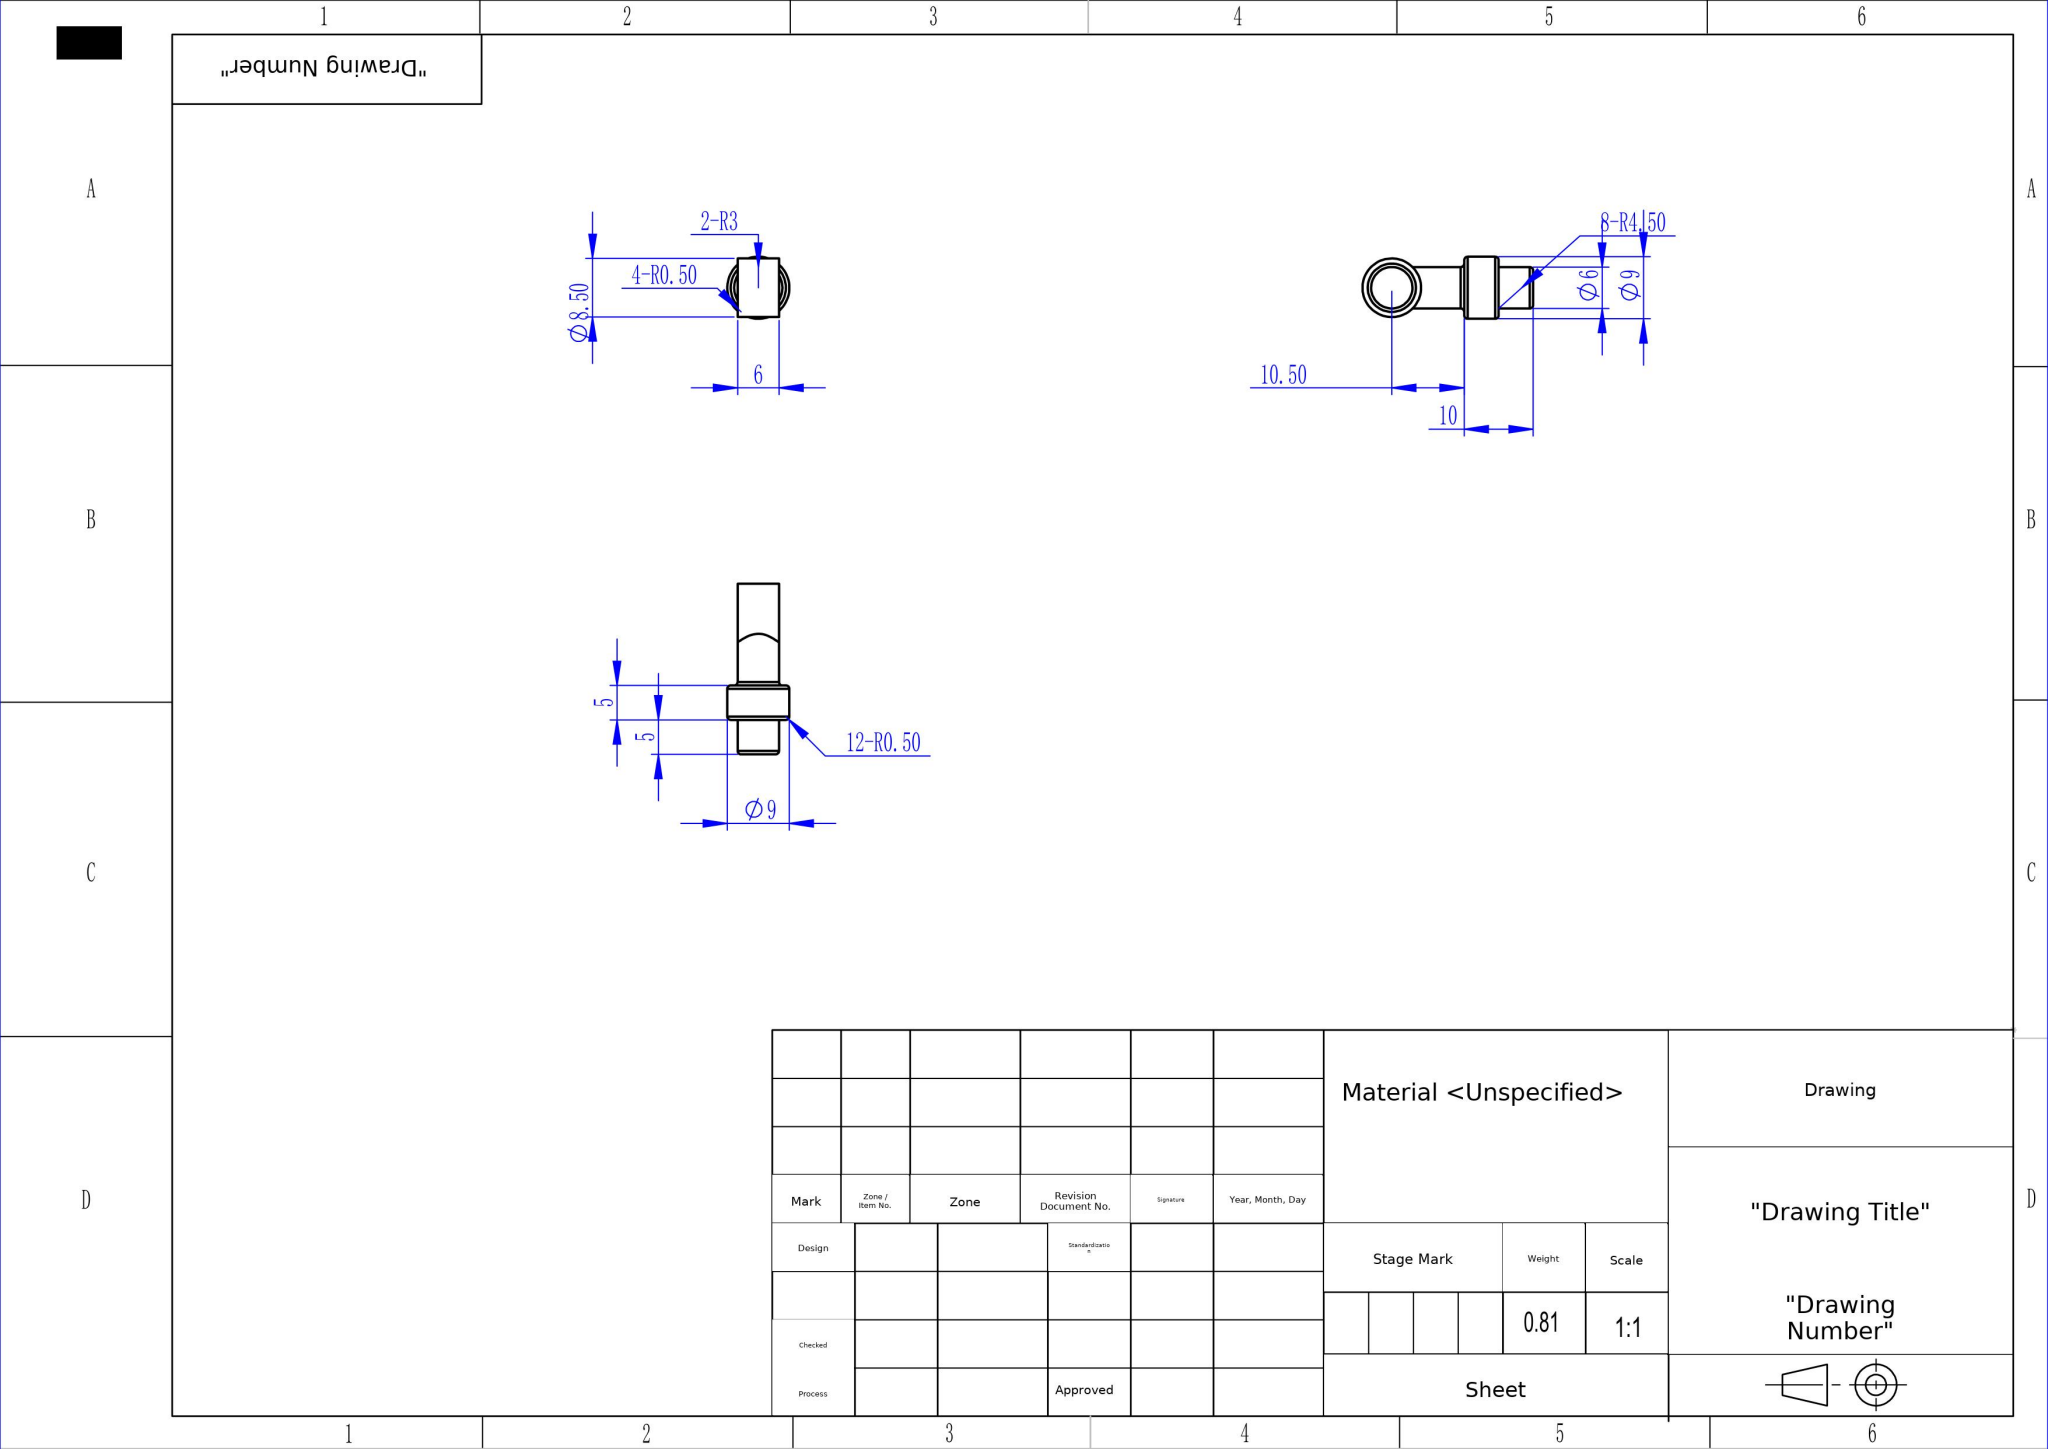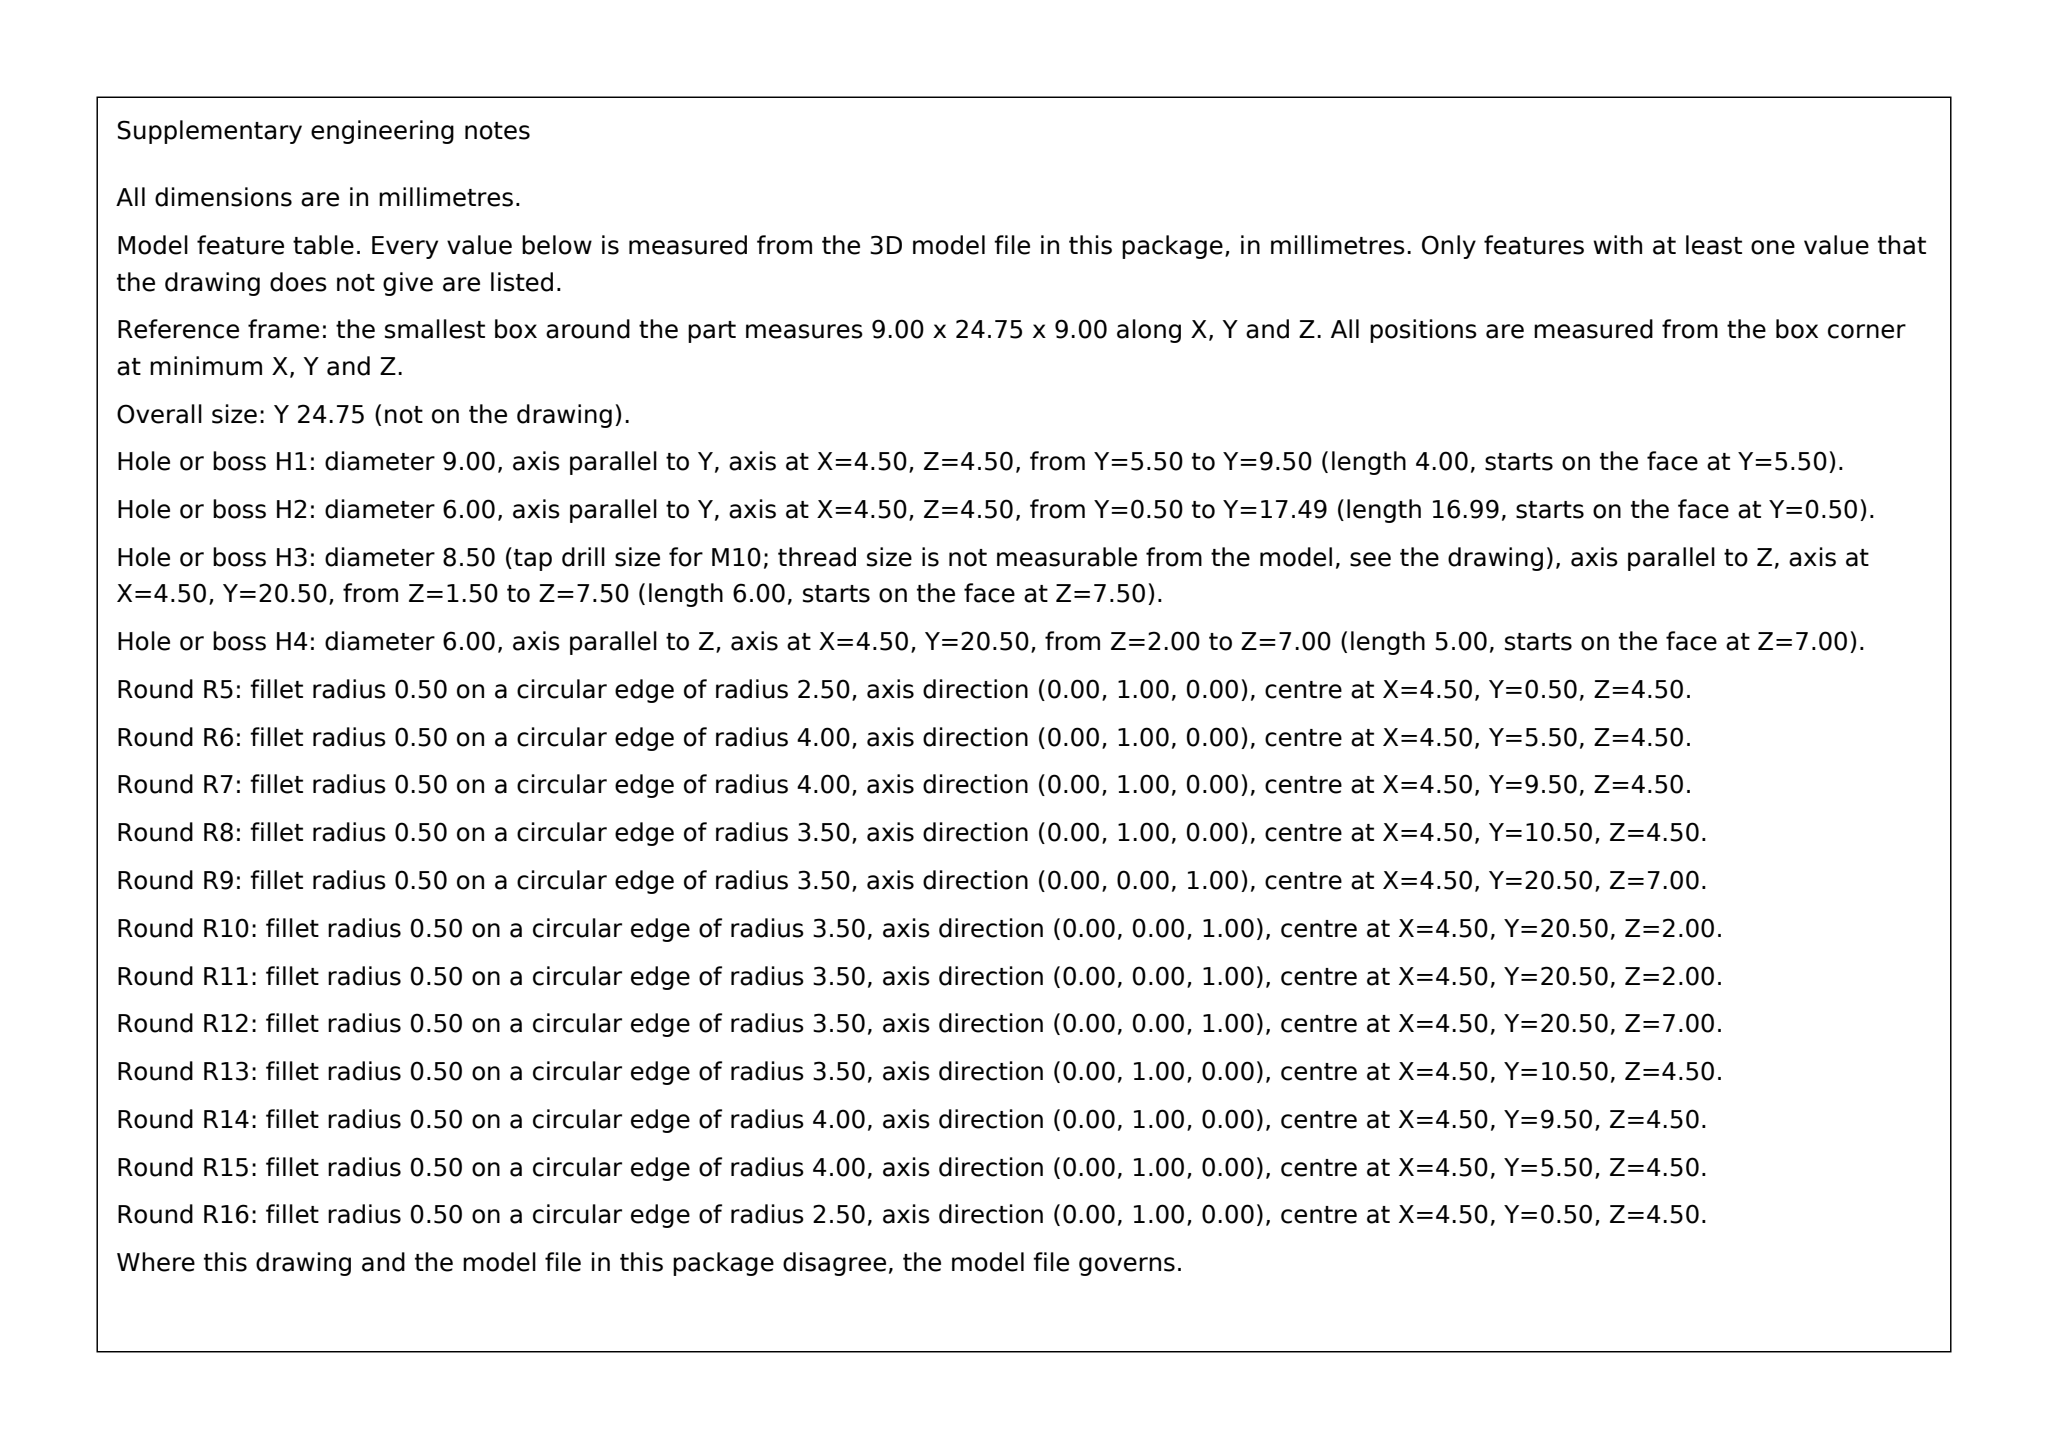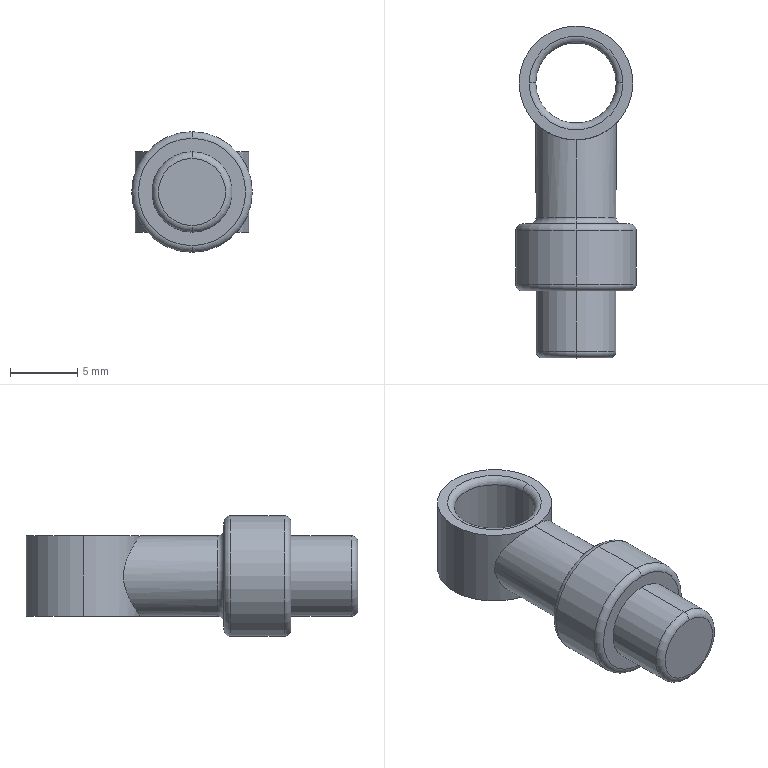Part | SolidWorks | mm | 1 solid | 28 faces | box 9 x 24.75 x 9 mm | volume 810 mm3 | torus 12 | cylinder 11 | plane 5 | commonest cylinder face diameters 6 x6 8.5 x3 9 x2
STEP:
#1=CARTESIAN_POINT('',(0.,0.,-2.5));
#2=VERTEX_POINT('',#1);
#3=CARTESIAN_POINT('',(0.,0.,2.5));
#4=VERTEX_POINT('',#3);
#5=CARTESIAN_POINT('',(0.,0.,0.));
#6=DIRECTION('',(0.,-1.,0.));
#7=DIRECTION('',(0.,0.,1.));
#8=AXIS2_PLACEMENT_3D('',#5,#6,#7);
#9=CIRCLE('',#8,2.5);
#10=EDGE_CURVE('',#2,#4,#9,.T.);
#11=ORIENTED_EDGE('',*,*,#10,.F.);
#12=CARTESIAN_POINT('',(0.,0.5,-3.));
#13=VERTEX_POINT('',#12);
#14=CARTESIAN_POINT('',(0.,0.5,-2.5));
#15=DIRECTION('',(1.,0.,0.));
#16=DIRECTION('',(0.,0.,-1.));
#17=AXIS2_PLACEMENT_3D('',#14,#15,#16);
#18=CIRCLE('',#17,0.5);
#19=EDGE_CURVE('',#2,#13,#18,.T.);
#20=ORIENTED_EDGE('',*,*,#19,.T.);
#21=CARTESIAN_POINT('',(0.,0.5,3.));
#22=VERTEX_POINT('',#21);
#23=CARTESIAN_POINT('',(0.,0.5,0.));
#24=DIRECTION('',(0.,1.,0.));
#25=DIRECTION('',(0.,0.,1.));
#26=AXIS2_PLACEMENT_3D('',#23,#24,#25);
#27=CIRCLE('',#26,3.);
#28=EDGE_CURVE('',#22,#13,#27,.T.);
#29=ORIENTED_EDGE('',*,*,#28,.F.);
#30=CARTESIAN_POINT('',(0.,0.5,2.5));
#31=DIRECTION('',(-1.,0.,0.));
#32=DIRECTION('',(0.,0.,1.));
#33=AXIS2_PLACEMENT_3D('',#30,#31,#32);
#34=CIRCLE('',#33,0.5);
#35=EDGE_CURVE('',#4,#22,#34,.T.);
#36=ORIENTED_EDGE('',*,*,#35,.F.);
#37=EDGE_LOOP('',(#11,#20,#29,#36));
#38=FACE_OUTER_BOUND('',#37,.T.);
#39=CARTESIAN_POINT('',(0.,0.5,0.));
#40=DIRECTION('',(0.,1.,0.));
#41=DIRECTION('',(0.,0.,1.));
#42=AXIS2_PLACEMENT_3D('',#39,#40,#41);
#43=TOROIDAL_SURFACE('',#42,2.5,0.5);
#44=ADVANCED_FACE('',(#38),#43,.T.);
#45=CARTESIAN_POINT('',(0.,5.,-4.));
#46=VERTEX_POINT('',#45);
#47=CARTESIAN_POINT('',(0.,5.,4.));
#48=VERTEX_POINT('',#47);
#49=CARTESIAN_POINT('',(0.,5.,0.));
#50=DIRECTION('',(0.,-1.,0.));
#51=DIRECTION('',(0.,0.,1.));
#52=AXIS2_PLACEMENT_3D('',#49,#50,#51);
#53=CIRCLE('',#52,4.);
#54=EDGE_CURVE('',#46,#48,#53,.T.);
#55=ORIENTED_EDGE('',*,*,#54,.F.);
#56=CARTESIAN_POINT('',(0.,5.5,-4.5));
#57=VERTEX_POINT('',#56);
#58=CARTESIAN_POINT('',(0.,5.5,-4.));
#59=DIRECTION('',(1.,0.,0.));
#60=DIRECTION('',(0.,0.,-1.));
#61=AXIS2_PLACEMENT_3D('',#58,#59,#60);
#62=CIRCLE('',#61,0.5);
#63=EDGE_CURVE('',#46,#57,#62,.T.);
#64=ORIENTED_EDGE('',*,*,#63,.T.);
#65=CARTESIAN_POINT('',(0.,5.5,4.5));
#66=VERTEX_POINT('',#65);
#67=CARTESIAN_POINT('',(0.,5.5,0.));
#68=DIRECTION('',(0.,1.,0.));
#69=DIRECTION('',(0.,0.,1.));
#70=AXIS2_PLACEMENT_3D('',#67,#68,#69);
#71=CIRCLE('',#70,4.5);
#72=EDGE_CURVE('',#66,#57,#71,.T.);
#73=ORIENTED_EDGE('',*,*,#72,.F.);
#74=CARTESIAN_POINT('',(0.,5.5,4.));
#75=DIRECTION('',(-1.,0.,0.));
#76=DIRECTION('',(0.,0.,1.));
#77=AXIS2_PLACEMENT_3D('',#74,#75,#76);
#78=CIRCLE('',#77,0.5);
#79=EDGE_CURVE('',#48,#66,#78,.T.);
#80=ORIENTED_EDGE('',*,*,#79,.F.);
#81=EDGE_LOOP('',(#55,#64,#73,#80));
#82=FACE_OUTER_BOUND('',#81,.T.);
#83=CARTESIAN_POINT('',(0.,5.5,0.));
#84=DIRECTION('',(0.,1.,0.));
#85=DIRECTION('',(0.,0.,1.));
#86=AXIS2_PLACEMENT_3D('',#83,#84,#85);
#87=TOROIDAL_SURFACE('',#86,4.,0.5);
#88=ADVANCED_FACE('',(#82),#87,.T.);
#89=CARTESIAN_POINT('',(0.,9.5,-4.5));
#90=VERTEX_POINT('',#89);
#91=CARTESIAN_POINT('',(0.,9.5,4.5));
#92=VERTEX_POINT('',#91);
#93=CARTESIAN_POINT('',(0.,9.5,0.));
#94=DIRECTION('',(0.,-1.,0.));
#95=DIRECTION('',(0.,0.,1.));
#96=AXIS2_PLACEMENT_3D('',#93,#94,#95);
#97=CIRCLE('',#96,4.5);
#98=EDGE_CURVE('',#90,#92,#97,.T.);
#99=ORIENTED_EDGE('',*,*,#98,.F.);
#100=CARTESIAN_POINT('',(0.,10.,-4.));
#101=VERTEX_POINT('',#100);
#102=CARTESIAN_POINT('',(0.,9.5,-4.));
#103=DIRECTION('',(1.,0.,0.));
#104=DIRECTION('',(0.,0.,-1.));
#105=AXIS2_PLACEMENT_3D('',#102,#103,#104);
#106=CIRCLE('',#105,0.5);
#107=EDGE_CURVE('',#90,#101,#106,.T.);
#108=ORIENTED_EDGE('',*,*,#107,.T.);
#109=CARTESIAN_POINT('',(0.,10.,4.));
#110=VERTEX_POINT('',#109);
#111=CARTESIAN_POINT('',(0.,10.,0.));
#112=DIRECTION('',(0.,1.,0.));
#113=DIRECTION('',(0.,0.,1.));
#114=AXIS2_PLACEMENT_3D('',#111,#112,#113);
#115=CIRCLE('',#114,4.);
#116=EDGE_CURVE('',#110,#101,#115,.T.);
#117=ORIENTED_EDGE('',*,*,#116,.F.);
#118=CARTESIAN_POINT('',(0.,9.5,4.));
#119=DIRECTION('',(-1.,0.,0.));
#120=DIRECTION('',(0.,0.,1.));
#121=AXIS2_PLACEMENT_3D('',#118,#119,#120);
#122=CIRCLE('',#121,0.5);
#123=EDGE_CURVE('',#92,#110,#122,.T.);
#124=ORIENTED_EDGE('',*,*,#123,.F.);
#125=EDGE_LOOP('',(#99,#108,#117,#124));
#126=FACE_OUTER_BOUND('',#125,.T.);
#127=CARTESIAN_POINT('',(0.,9.5,0.));
#128=DIRECTION('',(0.,1.,0.));
#129=DIRECTION('',(0.,0.,1.));
#130=AXIS2_PLACEMENT_3D('',#127,#128,#129);
#131=TOROIDAL_SURFACE('',#130,4.,0.5);
#132=ADVANCED_FACE('',(#126),#131,.T.);
#133=CARTESIAN_POINT('',(0.,10.5,-3.));
#134=VERTEX_POINT('',#133);
#135=CARTESIAN_POINT('',(0.,10.5,3.));
#136=VERTEX_POINT('',#135);
#137=CARTESIAN_POINT('',(0.,10.5,0.));
#138=DIRECTION('',(0.,1.,0.));
#139=DIRECTION('',(0.,0.,1.));
#140=AXIS2_PLACEMENT_3D('',#137,#138,#139);
#141=CIRCLE('',#140,3.);
#142=EDGE_CURVE('',#134,#136,#141,.T.);
#143=ORIENTED_EDGE('',*,*,#142,.F.);
#144=CARTESIAN_POINT('',(0.,10.,-3.5));
#145=VERTEX_POINT('',#144);
#146=CARTESIAN_POINT('',(0.,10.5,-3.5));
#147=DIRECTION('',(1.,0.,0.));
#148=DIRECTION('',(0.,0.,-1.));
#149=AXIS2_PLACEMENT_3D('',#146,#147,#148);
#150=CIRCLE('',#149,0.5);
#151=EDGE_CURVE('',#134,#145,#150,.T.);
#152=ORIENTED_EDGE('',*,*,#151,.T.);
#153=CARTESIAN_POINT('',(0.,10.,3.5));
#154=VERTEX_POINT('',#153);
#155=CARTESIAN_POINT('',(0.,10.,0.));
#156=DIRECTION('',(0.,-1.,0.));
#157=DIRECTION('',(0.,0.,1.));
#158=AXIS2_PLACEMENT_3D('',#155,#156,#157);
#159=CIRCLE('',#158,3.5);
#160=EDGE_CURVE('',#154,#145,#159,.T.);
#161=ORIENTED_EDGE('',*,*,#160,.F.);
#162=CARTESIAN_POINT('',(0.,10.5,3.5));
#163=DIRECTION('',(-1.,0.,0.));
#164=DIRECTION('',(0.,0.,1.));
#165=AXIS2_PLACEMENT_3D('',#162,#163,#164);
#166=CIRCLE('',#165,0.5);
#167=EDGE_CURVE('',#136,#154,#166,.T.);
#168=ORIENTED_EDGE('',*,*,#167,.F.);
#169=EDGE_LOOP('',(#143,#152,#161,#168));
#170=FACE_OUTER_BOUND('',#169,.T.);
#171=CARTESIAN_POINT('',(0.,10.5,0.));
#172=DIRECTION('',(0.,1.,0.));
#173=DIRECTION('',(0.,0.,1.));
#174=AXIS2_PLACEMENT_3D('',#171,#172,#173);
#175=TOROIDAL_SURFACE('',#174,3.5,0.5);
#176=ADVANCED_FACE('',(#170),#175,.F.);
#177=CARTESIAN_POINT('',(-3.5,20.5,3.));
#178=VERTEX_POINT('',#177);
#179=CARTESIAN_POINT('',(3.5,20.5,3.));
#180=VERTEX_POINT('',#179);
#181=CARTESIAN_POINT('',(0.,20.5,3.));
#182=DIRECTION('',(0.,0.,-1.));
#183=DIRECTION('',(1.,0.,0.));
#184=AXIS2_PLACEMENT_3D('',#181,#182,#183);
#185=CIRCLE('',#184,3.5);
#186=EDGE_CURVE('',#178,#180,#185,.T.);
#187=ORIENTED_EDGE('',*,*,#186,.F.);
#188=CARTESIAN_POINT('',(-3.,20.5,2.5));
#189=VERTEX_POINT('',#188);
#190=CARTESIAN_POINT('',(-3.5,20.5,2.5));
#191=DIRECTION('',(0.,1.,0.));
#192=DIRECTION('',(-1.,0.,0.));
#193=AXIS2_PLACEMENT_3D('',#190,#191,#192);
#194=CIRCLE('',#193,0.5);
#195=EDGE_CURVE('',#178,#189,#194,.T.);
#196=ORIENTED_EDGE('',*,*,#195,.T.);
#197=CARTESIAN_POINT('',(3.,20.5,2.5));
#198=VERTEX_POINT('',#197);
#199=CARTESIAN_POINT('',(0.,20.5,2.5));
#200=DIRECTION('',(0.,0.,1.));
#201=DIRECTION('',(1.,0.,0.));
#202=AXIS2_PLACEMENT_3D('',#199,#200,#201);
#203=CIRCLE('',#202,3.);
#204=EDGE_CURVE('',#198,#189,#203,.T.);
#205=ORIENTED_EDGE('',*,*,#204,.F.);
#206=CARTESIAN_POINT('',(3.5,20.5,2.5));
#207=DIRECTION('',(0.,-1.,0.));
#208=DIRECTION('',(0.,0.,-1.));
#209=AXIS2_PLACEMENT_3D('',#206,#207,#208);
#210=CIRCLE('',#209,0.5);
#211=EDGE_CURVE('',#180,#198,#210,.T.);
#212=ORIENTED_EDGE('',*,*,#211,.F.);
#213=EDGE_LOOP('',(#187,#196,#205,#212));
#214=FACE_OUTER_BOUND('',#213,.T.);
#215=CARTESIAN_POINT('',(0.,20.5,2.5));
#216=DIRECTION('',(0.,0.,1.));
#217=DIRECTION('',(1.,0.,0.));
#218=AXIS2_PLACEMENT_3D('',#215,#216,#217);
#219=TOROIDAL_SURFACE('',#218,3.5,0.5);
#220=ADVANCED_FACE('',(#214),#219,.T.);
#221=CARTESIAN_POINT('',(-3.,20.5,-2.5));
#222=VERTEX_POINT('',#221);
#223=CARTESIAN_POINT('',(3.,20.5,-2.5));
#224=VERTEX_POINT('',#223);
#225=CARTESIAN_POINT('',(0.,20.5,-2.5));
#226=DIRECTION('',(0.,0.,-1.));
#227=DIRECTION('',(1.,0.,0.));
#228=AXIS2_PLACEMENT_3D('',#225,#226,#227);
#229=CIRCLE('',#228,3.);
#230=EDGE_CURVE('',#222,#224,#229,.T.);
#231=ORIENTED_EDGE('',*,*,#230,.F.);
#232=CARTESIAN_POINT('',(-3.5,20.5,-3.));
#233=VERTEX_POINT('',#232);
#234=CARTESIAN_POINT('',(-3.5,20.5,-2.5));
#235=DIRECTION('',(0.,1.,0.));
#236=DIRECTION('',(-1.,0.,0.));
#237=AXIS2_PLACEMENT_3D('',#234,#235,#236);
#238=CIRCLE('',#237,0.5);
#239=EDGE_CURVE('',#222,#233,#238,.T.);
#240=ORIENTED_EDGE('',*,*,#239,.T.);
#241=CARTESIAN_POINT('',(3.5,20.5,-3.));
#242=VERTEX_POINT('',#241);
#243=CARTESIAN_POINT('',(0.,20.5,-3.));
#244=DIRECTION('',(0.,0.,1.));
#245=DIRECTION('',(1.,0.,0.));
#246=AXIS2_PLACEMENT_3D('',#243,#244,#245);
#247=CIRCLE('',#246,3.5);
#248=EDGE_CURVE('',#242,#233,#247,.T.);
#249=ORIENTED_EDGE('',*,*,#248,.F.);
#250=CARTESIAN_POINT('',(3.5,20.5,-2.5));
#251=DIRECTION('',(0.,-1.,0.));
#252=DIRECTION('',(0.,0.,-1.));
#253=AXIS2_PLACEMENT_3D('',#250,#251,#252);
#254=CIRCLE('',#253,0.5);
#255=EDGE_CURVE('',#224,#242,#254,.T.);
#256=ORIENTED_EDGE('',*,*,#255,.F.);
#257=EDGE_LOOP('',(#231,#240,#249,#256));
#258=FACE_OUTER_BOUND('',#257,.T.);
#259=CARTESIAN_POINT('',(0.,20.5,-2.5));
#260=DIRECTION('',(0.,0.,1.));
#261=DIRECTION('',(1.,0.,0.));
#262=AXIS2_PLACEMENT_3D('',#259,#260,#261);
#263=TOROIDAL_SURFACE('',#262,3.5,0.5);
#264=ADVANCED_FACE('',(#258),#263,.T.);
#265=CARTESIAN_POINT('',(0.,20.5,-2.5));
#266=DIRECTION('',(0.,0.,-1.));
#267=DIRECTION('',(1.,0.,0.));
#268=AXIS2_PLACEMENT_3D('',#265,#266,#267);
#269=CIRCLE('',#268,3.);
#270=EDGE_CURVE('',#224,#222,#269,.T.);
#271=ORIENTED_EDGE('',*,*,#270,.T.);
#272=CARTESIAN_POINT('',(-3.,20.5,-3.));
#273=DIRECTION('',(0.,0.,1.));
#274=VECTOR('',#273,1000.);
#275=LINE('',#272,#274);
#276=EDGE_CURVE('',#222,#189,#275,.T.);
#277=ORIENTED_EDGE('',*,*,#276,.T.);
#278=CARTESIAN_POINT('',(0.,20.5,2.5));
#279=DIRECTION('',(0.,0.,1.));
#280=DIRECTION('',(1.,0.,0.));
#281=AXIS2_PLACEMENT_3D('',#278,#279,#280);
#282=CIRCLE('',#281,3.);
#283=EDGE_CURVE('',#189,#198,#282,.T.);
#284=ORIENTED_EDGE('',*,*,#283,.T.);
#285=CARTESIAN_POINT('',(3.,20.5,-3.));
#286=DIRECTION('',(0.,0.,1.));
#287=VECTOR('',#286,1000.);
#288=LINE('',#285,#287);
#289=EDGE_CURVE('',#224,#198,#288,.T.);
#290=ORIENTED_EDGE('',*,*,#289,.F.);
#291=EDGE_LOOP('',(#271,#277,#284,#290));
#292=FACE_OUTER_BOUND('',#291,.T.);
#293=CARTESIAN_POINT('',(0.,20.5,-3.));
#294=DIRECTION('',(0.,0.,1.));
#295=DIRECTION('',(1.,0.,0.));
#296=AXIS2_PLACEMENT_3D('',#293,#294,#295);
#297=CYLINDRICAL_SURFACE('',#296,3.);
#298=ADVANCED_FACE('',(#292),#297,.F.);
#299=CARTESIAN_POINT('',(4.25,20.5,-3.));
#300=VERTEX_POINT('',#299);
#301=CARTESIAN_POINT('',(-4.25,20.5,-3.));
#302=VERTEX_POINT('',#301);
#303=CARTESIAN_POINT('',(0.,20.5,-3.));
#304=DIRECTION('',(0.,0.,1.));
#305=DIRECTION('',(1.,0.,0.));
#306=AXIS2_PLACEMENT_3D('',#303,#304,#305);
#307=CIRCLE('',#306,4.25);
#308=EDGE_CURVE('',#300,#302,#307,.T.);
#309=ORIENTED_EDGE('',*,*,#308,.T.);
#310=CARTESIAN_POINT('',(-4.25,20.5,3.));
#311=VERTEX_POINT('',#310);
#312=CARTESIAN_POINT('',(-4.25,20.5,-3.));
#313=DIRECTION('',(0.,0.,1.));
#314=VECTOR('',#313,1000.);
#315=LINE('',#312,#314);
#316=EDGE_CURVE('',#302,#311,#315,.T.);
#317=ORIENTED_EDGE('',*,*,#316,.T.);
#318=CARTESIAN_POINT('',(4.25,20.5,3.));
#319=VERTEX_POINT('',#318);
#320=CARTESIAN_POINT('',(0.,20.5,3.));
#321=DIRECTION('',(0.,0.,1.));
#322=DIRECTION('',(1.,0.,0.));
#323=AXIS2_PLACEMENT_3D('',#320,#321,#322);
#324=CIRCLE('',#323,4.25);
#325=EDGE_CURVE('',#319,#311,#324,.T.);
#326=ORIENTED_EDGE('',*,*,#325,.F.);
#327=CARTESIAN_POINT('',(4.25,20.5,-3.));
#328=DIRECTION('',(0.,0.,1.));
#329=VECTOR('',#328,1000.);
#330=LINE('',#327,#329);
#331=EDGE_CURVE('',#300,#319,#330,.T.);
#332=ORIENTED_EDGE('',*,*,#331,.F.);
#333=EDGE_LOOP('',(#309,#317,#326,#332));
#334=FACE_OUTER_BOUND('',#333,.T.);
#335=CARTESIAN_POINT('',(0.,20.5,-3.));
#336=DIRECTION('',(0.,0.,1.));
#337=DIRECTION('',(1.,0.,0.));
#338=AXIS2_PLACEMENT_3D('',#335,#336,#337);
#339=CYLINDRICAL_SURFACE('',#338,4.25);
#340=ADVANCED_FACE('',(#334),#339,.T.);
#341=CARTESIAN_POINT('',(0.,16.25,-3.));
#342=VERTEX_POINT('',#341);
#343=CARTESIAN_POINT('',(0.,20.5,-3.));
#344=DIRECTION('',(0.,0.,1.));
#345=DIRECTION('',(1.,0.,0.));
#346=AXIS2_PLACEMENT_3D('',#343,#344,#345);
#347=CIRCLE('',#346,4.25);
#348=EDGE_CURVE('',#342,#300,#347,.T.);
#349=ORIENTED_EDGE('',*,*,#348,.T.);
#350=ORIENTED_EDGE('',*,*,#331,.T.);
#351=CARTESIAN_POINT('',(0.,16.25,3.));
#352=VERTEX_POINT('',#351);
#353=CARTESIAN_POINT('',(0.,20.5,3.));
#354=DIRECTION('',(0.,0.,1.));
#355=DIRECTION('',(1.,0.,0.));
#356=AXIS2_PLACEMENT_3D('',#353,#354,#355);
#357=CIRCLE('',#356,4.25);
#358=EDGE_CURVE('',#352,#319,#357,.T.);
#359=ORIENTED_EDGE('',*,*,#358,.F.);
#360=CARTESIAN_POINT('',(0.,16.25,-3.));
#361=CARTESIAN_POINT('',(0.2066,16.25,-3.));
#362=CARTESIAN_POINT('',(0.4085,16.265,-2.979));
#363=CARTESIAN_POINT('',(0.8037,16.322,-2.897));
#364=CARTESIAN_POINT('',(0.9982,16.365,-2.836));
#365=CARTESIAN_POINT('',(1.361,16.469,-2.681));
#366=CARTESIAN_POINT('',(1.532,16.532,-2.587));
#367=CARTESIAN_POINT('',(1.852,16.671,-2.368));
#368=CARTESIAN_POINT('',(1.997,16.745,-2.246));
#369=CARTESIAN_POINT('',(2.264,16.9,-1.978));
#370=CARTESIAN_POINT('',(2.385,16.98,-1.83));
#371=CARTESIAN_POINT('',(2.596,17.132,-1.516));
#372=CARTESIAN_POINT('',(2.686,17.205,-1.35));
#373=CARTESIAN_POINT('',(2.838,17.334,-0.9929));
#374=CARTESIAN_POINT('',(2.898,17.391,-0.8018));
#375=CARTESIAN_POINT('',(2.979,17.468,-0.4093));
#376=CARTESIAN_POINT('',(3.,17.49,-0.2024));
#377=CARTESIAN_POINT('',(3.,17.489,0.2058));
#378=CARTESIAN_POINT('',(2.979,17.468,0.4094));
#379=CARTESIAN_POINT('',(2.897,17.39,0.8053));
#380=CARTESIAN_POINT('',(2.838,17.335,0.9924));
#381=CARTESIAN_POINT('',(2.686,17.205,1.35));
#382=CARTESIAN_POINT('',(2.594,17.131,1.52));
#383=CARTESIAN_POINT('',(2.383,16.978,1.833));
#384=CARTESIAN_POINT('',(2.264,16.9,1.978));
#385=CARTESIAN_POINT('',(1.997,16.745,2.247));
#386=CARTESIAN_POINT('',(1.849,16.669,2.37));
#387=CARTESIAN_POINT('',(1.534,16.533,2.585));
#388=CARTESIAN_POINT('',(1.364,16.471,2.679));
#389=CARTESIAN_POINT('',(0.9995,16.365,2.836));
#390=CARTESIAN_POINT('',(0.8069,16.323,2.897));
#391=CARTESIAN_POINT('',(0.4114,16.265,2.979));
#392=CARTESIAN_POINT('',(0.2041,16.25,3.));
#393=CARTESIAN_POINT('',(0.,16.25,3.));
#394=B_SPLINE_CURVE_WITH_KNOTS('',3,(#360,#361,#362,#363,#364,#365,#366,#367,#368,#369,#370,#371,#372,#373,#374,#375,#376,#377,#378,#379,#380,#381,#382,#383,#384,#385,#386,#387,#388,#389,#390,#391,#392,#393),.UNSPECIFIED.,.F.,.F.,(4,2,2,2,2,2,2,2,2,2,2,2,2,2,2,2,4),(0.,0.0006099,0.00122,0.00183,0.002439,0.003049,0.003659,0.004269,0.004879,0.005489,0.006099,0.006709,0.007318,0.007928,0.008538,0.009148,0.009758),.UNSPECIFIED.);
#395=EDGE_CURVE('',#342,#352,#394,.T.);
#396=ORIENTED_EDGE('',*,*,#395,.F.);
#397=EDGE_LOOP('',(#349,#350,#359,#396));
#398=FACE_OUTER_BOUND('',#397,.T.);
#399=CARTESIAN_POINT('',(0.,20.5,-3.));
#400=DIRECTION('',(0.,0.,1.));
#401=DIRECTION('',(1.,0.,0.));
#402=AXIS2_PLACEMENT_3D('',#399,#400,#401);
#403=CYLINDRICAL_SURFACE('',#402,4.25);
#404=ADVANCED_FACE('',(#398),#403,.T.);
#405=ORIENTED_EDGE('',*,*,#395,.T.);
#406=CARTESIAN_POINT('',(0.,17.5,3.));
#407=DIRECTION('',(0.,-1.,0.));
#408=VECTOR('',#407,1000.);
#409=LINE('',#406,#408);
#410=EDGE_CURVE('',#352,#136,#409,.T.);
#411=ORIENTED_EDGE('',*,*,#410,.T.);
#412=CARTESIAN_POINT('',(0.,10.5,0.));
#413=DIRECTION('',(0.,1.,0.));
#414=DIRECTION('',(0.,0.,1.));
#415=AXIS2_PLACEMENT_3D('',#412,#413,#414);
#416=CIRCLE('',#415,3.);
#417=EDGE_CURVE('',#136,#134,#416,.T.);
#418=ORIENTED_EDGE('',*,*,#417,.T.);
#419=CARTESIAN_POINT('',(0.,17.5,-3.));
#420=DIRECTION('',(0.,-1.,0.));
#421=VECTOR('',#420,1000.);
#422=LINE('',#419,#421);
#423=EDGE_CURVE('',#342,#134,#422,.T.);
#424=ORIENTED_EDGE('',*,*,#423,.F.);
#425=EDGE_LOOP('',(#405,#411,#418,#424));
#426=FACE_OUTER_BOUND('',#425,.T.);
#427=CARTESIAN_POINT('',(0.,17.5,0.));
#428=DIRECTION('',(0.,-1.,0.));
#429=DIRECTION('',(0.,0.,-1.));
#430=AXIS2_PLACEMENT_3D('',#427,#428,#429);
#431=CYLINDRICAL_SURFACE('',#430,3.);
#432=ADVANCED_FACE('',(#426),#431,.T.);
#433=ORIENTED_EDGE('',*,*,#98,.T.);
#434=CARTESIAN_POINT('',(0.,10.,4.5));
#435=DIRECTION('',(0.,-1.,0.));
#436=VECTOR('',#435,1000.);
#437=LINE('',#434,#436);
#438=EDGE_CURVE('',#92,#66,#437,.T.);
#439=ORIENTED_EDGE('',*,*,#438,.T.);
#440=ORIENTED_EDGE('',*,*,#72,.T.);
#441=CARTESIAN_POINT('',(0.,10.,-4.5));
#442=DIRECTION('',(0.,-1.,0.));
#443=VECTOR('',#442,1000.);
#444=LINE('',#441,#443);
#445=EDGE_CURVE('',#90,#57,#444,.T.);
#446=ORIENTED_EDGE('',*,*,#445,.F.);
#447=EDGE_LOOP('',(#433,#439,#440,#446));
#448=FACE_OUTER_BOUND('',#447,.T.);
#449=CARTESIAN_POINT('',(0.,10.,0.));
#450=DIRECTION('',(0.,-1.,0.));
#451=DIRECTION('',(0.,0.,-1.));
#452=AXIS2_PLACEMENT_3D('',#449,#450,#451);
#453=CYLINDRICAL_SURFACE('',#452,4.5);
#454=ADVANCED_FACE('',(#448),#453,.T.);
#455=CARTESIAN_POINT('',(0.,5.,3.));
#456=VERTEX_POINT('',#455);
#457=CARTESIAN_POINT('',(0.,5.,-3.));
#458=VERTEX_POINT('',#457);
#459=CARTESIAN_POINT('',(0.,5.,0.));
#460=DIRECTION('',(0.,1.,0.));
#461=DIRECTION('',(0.,0.,1.));
#462=AXIS2_PLACEMENT_3D('',#459,#460,#461);
#463=CIRCLE('',#462,3.);
#464=EDGE_CURVE('',#456,#458,#463,.T.);
#465=ORIENTED_EDGE('',*,*,#464,.F.);
#466=CARTESIAN_POINT('',(0.,5.,3.));
#467=DIRECTION('',(0.,-1.,0.));
#468=VECTOR('',#467,1000.);
#469=LINE('',#466,#468);
#470=EDGE_CURVE('',#456,#22,#469,.T.);
#471=ORIENTED_EDGE('',*,*,#470,.T.);
#472=ORIENTED_EDGE('',*,*,#28,.T.);
#473=CARTESIAN_POINT('',(0.,5.,-3.));
#474=DIRECTION('',(0.,-1.,0.));
#475=VECTOR('',#474,1000.);
#476=LINE('',#473,#475);
#477=EDGE_CURVE('',#458,#13,#476,.T.);
#478=ORIENTED_EDGE('',*,*,#477,.F.);
#479=EDGE_LOOP('',(#465,#471,#472,#478));
#480=FACE_OUTER_BOUND('',#479,.T.);
#481=CARTESIAN_POINT('',(0.,5.,0.));
#482=DIRECTION('',(0.,-1.,0.));
#483=DIRECTION('',(0.,0.,-1.));
#484=AXIS2_PLACEMENT_3D('',#481,#482,#483);
#485=CYLINDRICAL_SURFACE('',#484,3.);
#486=ADVANCED_FACE('',(#480),#485,.T.);
#487=ORIENTED_EDGE('',*,*,#470,.F.);
#488=CARTESIAN_POINT('',(0.,5.,0.));
#489=DIRECTION('',(0.,1.,0.));
#490=DIRECTION('',(0.,0.,1.));
#491=AXIS2_PLACEMENT_3D('',#488,#489,#490);
#492=CIRCLE('',#491,3.);
#493=EDGE_CURVE('',#458,#456,#492,.T.);
#494=ORIENTED_EDGE('',*,*,#493,.F.);
#495=ORIENTED_EDGE('',*,*,#477,.T.);
#496=CARTESIAN_POINT('',(0.,0.5,0.));
#497=DIRECTION('',(0.,1.,0.));
#498=DIRECTION('',(0.,0.,1.));
#499=AXIS2_PLACEMENT_3D('',#496,#497,#498);
#500=CIRCLE('',#499,3.);
#501=EDGE_CURVE('',#13,#22,#500,.T.);
#502=ORIENTED_EDGE('',*,*,#501,.T.);
#503=EDGE_LOOP('',(#487,#494,#495,#502));
#504=FACE_OUTER_BOUND('',#503,.T.);
#505=CARTESIAN_POINT('',(0.,5.,0.));
#506=DIRECTION('',(0.,-1.,0.));
#507=DIRECTION('',(0.,0.,-1.));
#508=AXIS2_PLACEMENT_3D('',#505,#506,#507);
#509=CYLINDRICAL_SURFACE('',#508,3.);
#510=ADVANCED_FACE('',(#504),#509,.T.);
#511=CARTESIAN_POINT('',(0.,0.,0.));
#512=DIRECTION('',(0.,-1.,0.));
#513=DIRECTION('',(0.,0.,1.));
#514=AXIS2_PLACEMENT_3D('',#511,#512,#513);
#515=CIRCLE('',#514,2.5);
#516=EDGE_CURVE('',#4,#2,#515,.T.);
#517=ORIENTED_EDGE('',*,*,#516,.T.);
#518=ORIENTED_EDGE('',*,*,#10,.T.);
#519=EDGE_LOOP('',(#517,#518));
#520=FACE_OUTER_BOUND('',#519,.T.);
#521=CARTESIAN_POINT('',(0.,0.,0.));
#522=DIRECTION('',(0.,1.,0.));
#523=DIRECTION('',(0.,0.,1.));
#524=AXIS2_PLACEMENT_3D('',#521,#522,#523);
#525=PLANE('',#524);
#526=ADVANCED_FACE('',(#520),#525,.F.);
#527=ORIENTED_EDGE('',*,*,#438,.F.);
#528=CARTESIAN_POINT('',(0.,9.5,0.));
#529=DIRECTION('',(0.,-1.,0.));
#530=DIRECTION('',(0.,0.,1.));
#531=AXIS2_PLACEMENT_3D('',#528,#529,#530);
#532=CIRCLE('',#531,4.5);
#533=EDGE_CURVE('',#92,#90,#532,.T.);
#534=ORIENTED_EDGE('',*,*,#533,.T.);
#535=ORIENTED_EDGE('',*,*,#445,.T.);
#536=CARTESIAN_POINT('',(0.,5.5,0.));
#537=DIRECTION('',(0.,1.,0.));
#538=DIRECTION('',(0.,0.,1.));
#539=AXIS2_PLACEMENT_3D('',#536,#537,#538);
#540=CIRCLE('',#539,4.5);
#541=EDGE_CURVE('',#57,#66,#540,.T.);
#542=ORIENTED_EDGE('',*,*,#541,.T.);
#543=EDGE_LOOP('',(#527,#534,#535,#542));
#544=FACE_OUTER_BOUND('',#543,.T.);
#545=CARTESIAN_POINT('',(0.,10.,0.));
#546=DIRECTION('',(0.,-1.,0.));
#547=DIRECTION('',(0.,0.,-1.));
#548=AXIS2_PLACEMENT_3D('',#545,#546,#547);
#549=CYLINDRICAL_SURFACE('',#548,4.5);
#550=ADVANCED_FACE('',(#544),#549,.T.);
#551=ORIENTED_EDGE('',*,*,#160,.T.);
#552=CARTESIAN_POINT('',(0.,10.,0.));
#553=DIRECTION('',(0.,-1.,0.));
#554=DIRECTION('',(0.,0.,1.));
#555=AXIS2_PLACEMENT_3D('',#552,#553,#554);
#556=CIRCLE('',#555,3.5);
#557=EDGE_CURVE('',#145,#154,#556,.T.);
#558=ORIENTED_EDGE('',*,*,#557,.T.);
#559=EDGE_LOOP('',(#551,#558));
#560=FACE_BOUND('',#559,.T.);
#561=ORIENTED_EDGE('',*,*,#116,.T.);
#562=CARTESIAN_POINT('',(0.,10.,0.));
#563=DIRECTION('',(0.,1.,0.));
#564=DIRECTION('',(0.,0.,1.));
#565=AXIS2_PLACEMENT_3D('',#562,#563,#564);
#566=CIRCLE('',#565,4.);
#567=EDGE_CURVE('',#101,#110,#566,.T.);
#568=ORIENTED_EDGE('',*,*,#567,.T.);
#569=EDGE_LOOP('',(#561,#568));
#570=FACE_OUTER_BOUND('',#569,.T.);
#571=CARTESIAN_POINT('',(0.,10.,0.));
#572=DIRECTION('',(0.,1.,0.));
#573=DIRECTION('',(0.,0.,1.));
#574=AXIS2_PLACEMENT_3D('',#571,#572,#573);
#575=PLANE('',#574);
#576=ADVANCED_FACE('',(#560,#570),#575,.T.);
#577=CARTESIAN_POINT('',(0.,5.,0.));
#578=DIRECTION('',(0.,-1.,0.));
#579=DIRECTION('',(0.,0.,1.));
#580=AXIS2_PLACEMENT_3D('',#577,#578,#579);
#581=CIRCLE('',#580,4.);
#582=EDGE_CURVE('',#48,#46,#581,.T.);
#583=ORIENTED_EDGE('',*,*,#582,.T.);
#584=ORIENTED_EDGE('',*,*,#54,.T.);
#585=EDGE_LOOP('',(#583,#584));
#586=FACE_OUTER_BOUND('',#585,.T.);
#587=ORIENTED_EDGE('',*,*,#493,.T.);
#588=ORIENTED_EDGE('',*,*,#464,.T.);
#589=EDGE_LOOP('',(#587,#588));
#590=FACE_BOUND('',#589,.T.);
#591=CARTESIAN_POINT('',(0.,5.,0.));
#592=DIRECTION('',(0.,1.,0.));
#593=DIRECTION('',(0.,0.,1.));
#594=AXIS2_PLACEMENT_3D('',#591,#592,#593);
#595=PLANE('',#594);
#596=ADVANCED_FACE('',(#586,#590),#595,.F.);
#597=ORIENTED_EDGE('',*,*,#410,.F.);
#598=CARTESIAN_POINT('',(0.,16.25,3.));
#599=CARTESIAN_POINT('',(-0.2036,16.25,3.));
#600=CARTESIAN_POINT('',(-0.4061,16.265,2.979));
#601=CARTESIAN_POINT('',(-0.8059,16.322,2.897));
#602=CARTESIAN_POINT('',(-0.9961,16.364,2.837));
#603=CARTESIAN_POINT('',(-1.36,16.469,2.681));
#604=CARTESIAN_POINT('',(-1.533,16.532,2.586));
#605=CARTESIAN_POINT('',(-1.85,16.67,2.37));
#606=CARTESIAN_POINT('',(-1.997,16.745,2.247));
#607=CARTESIAN_POINT('',(-2.264,16.9,1.977));
#608=CARTESIAN_POINT('',(-2.383,16.979,1.832));
#609=CARTESIAN_POINT('',(-2.594,17.131,1.519));
#610=CARTESIAN_POINT('',(-2.687,17.206,1.349));
#611=CARTESIAN_POINT('',(-2.838,17.335,0.9921));
#612=CARTESIAN_POINT('',(-2.897,17.39,0.8051));
#613=CARTESIAN_POINT('',(-2.979,17.468,0.4081));
#614=CARTESIAN_POINT('',(-3.,17.49,0.2062));
#615=CARTESIAN_POINT('',(-3.,17.49,-0.2037));
#616=CARTESIAN_POINT('',(-2.979,17.468,-0.409));
#617=CARTESIAN_POINT('',(-2.898,17.391,-0.8018));
#618=CARTESIAN_POINT('',(-2.837,17.334,-0.993));
#619=CARTESIAN_POINT('',(-2.611,17.141,-1.526));
#620=CARTESIAN_POINT('',(-2.396,16.977,-1.844));
#621=CARTESIAN_POINT('',(-1.998,16.746,-2.246));
#622=CARTESIAN_POINT('',(-1.85,16.67,-2.369));
#623=CARTESIAN_POINT('',(-1.532,16.532,-2.586));
#624=CARTESIAN_POINT('',(-1.363,16.47,-2.68));
#625=CARTESIAN_POINT('',(-0.9999,16.365,-2.835));
#626=CARTESIAN_POINT('',(-0.8059,16.322,-2.897));
#627=CARTESIAN_POINT('',(-0.4113,16.265,-2.979));
#628=CARTESIAN_POINT('',(-0.2062,16.25,-3.));
#629=CARTESIAN_POINT('',(0.,16.25,-3.));
#630=B_SPLINE_CURVE_WITH_KNOTS('',3,(#598,#599,#600,#601,#602,#603,#604,#605,#606,#607,#608,#609,#610,#611,#612,#613,#614,#615,#616,#617,#618,#619,#620,#621,#622,#623,#624,#625,#626,#627,#628,#629),.UNSPECIFIED.,.F.,.F.,(4,2,2,2,2,2,2,2,2,2,2,2,2,2,2,4),(0.009758,0.01037,0.01098,0.01158,0.01219,0.0128,0.01341,0.01402,0.01463,0.01524,0.01584,0.01706,0.01767,0.01828,0.01889,0.0195),.UNSPECIFIED.);
#631=EDGE_CURVE('',#352,#342,#630,.T.);
#632=ORIENTED_EDGE('',*,*,#631,.T.);
#633=ORIENTED_EDGE('',*,*,#423,.T.);
#634=ORIENTED_EDGE('',*,*,#142,.T.);
#635=EDGE_LOOP('',(#597,#632,#633,#634));
#636=FACE_OUTER_BOUND('',#635,.T.);
#637=CARTESIAN_POINT('',(0.,17.5,0.));
#638=DIRECTION('',(0.,-1.,0.));
#639=DIRECTION('',(0.,0.,-1.));
#640=AXIS2_PLACEMENT_3D('',#637,#638,#639);
#641=CYLINDRICAL_SURFACE('',#640,3.);
#642=ADVANCED_FACE('',(#636),#641,.T.);
#643=ORIENTED_EDGE('',*,*,#316,.F.);
#644=CARTESIAN_POINT('',(0.,20.5,-3.));
#645=DIRECTION('',(0.,0.,1.));
#646=DIRECTION('',(1.,0.,0.));
#647=AXIS2_PLACEMENT_3D('',#644,#645,#646);
#648=CIRCLE('',#647,4.25);
#649=EDGE_CURVE('',#302,#342,#648,.T.);
#650=ORIENTED_EDGE('',*,*,#649,.T.);
#651=ORIENTED_EDGE('',*,*,#631,.F.);
#652=CARTESIAN_POINT('',(0.,20.5,3.));
#653=DIRECTION('',(0.,0.,1.));
#654=DIRECTION('',(1.,0.,0.));
#655=AXIS2_PLACEMENT_3D('',#652,#653,#654);
#656=CIRCLE('',#655,4.25);
#657=EDGE_CURVE('',#311,#352,#656,.T.);
#658=ORIENTED_EDGE('',*,*,#657,.F.);
#659=EDGE_LOOP('',(#643,#650,#651,#658));
#660=FACE_OUTER_BOUND('',#659,.T.);
#661=CARTESIAN_POINT('',(0.,20.5,-3.));
#662=DIRECTION('',(0.,0.,1.));
#663=DIRECTION('',(1.,0.,0.));
#664=AXIS2_PLACEMENT_3D('',#661,#662,#663);
#665=CYLINDRICAL_SURFACE('',#664,4.25);
#666=ADVANCED_FACE('',(#660),#665,.T.);
#667=ORIENTED_EDGE('',*,*,#248,.T.);
#668=CARTESIAN_POINT('',(0.,20.5,-3.));
#669=DIRECTION('',(0.,0.,1.));
#670=DIRECTION('',(1.,0.,0.));
#671=AXIS2_PLACEMENT_3D('',#668,#669,#670);
#672=CIRCLE('',#671,3.5);
#673=EDGE_CURVE('',#233,#242,#672,.T.);
#674=ORIENTED_EDGE('',*,*,#673,.T.);
#675=EDGE_LOOP('',(#667,#674));
#676=FACE_BOUND('',#675,.T.);
#677=ORIENTED_EDGE('',*,*,#348,.F.);
#678=ORIENTED_EDGE('',*,*,#649,.F.);
#679=ORIENTED_EDGE('',*,*,#308,.F.);
#680=EDGE_LOOP('',(#677,#678,#679));
#681=FACE_OUTER_BOUND('',#680,.T.);
#682=CARTESIAN_POINT('',(0.,20.5,-3.));
#683=DIRECTION('',(0.,0.,1.));
#684=DIRECTION('',(1.,0.,0.));
#685=AXIS2_PLACEMENT_3D('',#682,#683,#684);
#686=PLANE('',#685);
#687=ADVANCED_FACE('',(#676,#681),#686,.F.);
#688=ORIENTED_EDGE('',*,*,#276,.F.);
#689=ORIENTED_EDGE('',*,*,#230,.T.);
#690=ORIENTED_EDGE('',*,*,#289,.T.);
#691=ORIENTED_EDGE('',*,*,#204,.T.);
#692=EDGE_LOOP('',(#688,#689,#690,#691));
#693=FACE_OUTER_BOUND('',#692,.T.);
#694=CARTESIAN_POINT('',(0.,20.5,-3.));
#695=DIRECTION('',(0.,0.,1.));
#696=DIRECTION('',(1.,0.,0.));
#697=AXIS2_PLACEMENT_3D('',#694,#695,#696);
#698=CYLINDRICAL_SURFACE('',#697,3.);
#699=ADVANCED_FACE('',(#693),#698,.F.);
#700=CARTESIAN_POINT('',(0.,20.5,3.));
#701=DIRECTION('',(0.,0.,-1.));
#702=DIRECTION('',(1.,0.,0.));
#703=AXIS2_PLACEMENT_3D('',#700,#701,#702);
#704=CIRCLE('',#703,3.5);
#705=EDGE_CURVE('',#180,#178,#704,.T.);
#706=ORIENTED_EDGE('',*,*,#705,.T.);
#707=ORIENTED_EDGE('',*,*,#186,.T.);
#708=EDGE_LOOP('',(#706,#707));
#709=FACE_BOUND('',#708,.T.);
#710=ORIENTED_EDGE('',*,*,#358,.T.);
#711=ORIENTED_EDGE('',*,*,#325,.T.);
#712=ORIENTED_EDGE('',*,*,#657,.T.);
#713=EDGE_LOOP('',(#710,#711,#712));
#714=FACE_OUTER_BOUND('',#713,.T.);
#715=CARTESIAN_POINT('',(0.,20.5,3.));
#716=DIRECTION('',(0.,0.,1.));
#717=DIRECTION('',(1.,0.,0.));
#718=AXIS2_PLACEMENT_3D('',#715,#716,#717);
#719=PLANE('',#718);
#720=ADVANCED_FACE('',(#709,#714),#719,.T.);
#721=ORIENTED_EDGE('',*,*,#239,.F.);
#722=ORIENTED_EDGE('',*,*,#270,.F.);
#723=ORIENTED_EDGE('',*,*,#255,.T.);
#724=ORIENTED_EDGE('',*,*,#673,.F.);
#725=EDGE_LOOP('',(#721,#722,#723,#724));
#726=FACE_OUTER_BOUND('',#725,.T.);
#727=CARTESIAN_POINT('',(0.,20.5,-2.5));
#728=DIRECTION('',(0.,0.,1.));
#729=DIRECTION('',(1.,0.,0.));
#730=AXIS2_PLACEMENT_3D('',#727,#728,#729);
#731=TOROIDAL_SURFACE('',#730,3.5,0.5);
#732=ADVANCED_FACE('',(#726),#731,.T.);
#733=ORIENTED_EDGE('',*,*,#195,.F.);
#734=ORIENTED_EDGE('',*,*,#705,.F.);
#735=ORIENTED_EDGE('',*,*,#211,.T.);
#736=ORIENTED_EDGE('',*,*,#283,.F.);
#737=EDGE_LOOP('',(#733,#734,#735,#736));
#738=FACE_OUTER_BOUND('',#737,.T.);
#739=CARTESIAN_POINT('',(0.,20.5,2.5));
#740=DIRECTION('',(0.,0.,1.));
#741=DIRECTION('',(1.,0.,0.));
#742=AXIS2_PLACEMENT_3D('',#739,#740,#741);
#743=TOROIDAL_SURFACE('',#742,3.5,0.5);
#744=ADVANCED_FACE('',(#738),#743,.T.);
#745=ORIENTED_EDGE('',*,*,#151,.F.);
#746=ORIENTED_EDGE('',*,*,#417,.F.);
#747=ORIENTED_EDGE('',*,*,#167,.T.);
#748=ORIENTED_EDGE('',*,*,#557,.F.);
#749=EDGE_LOOP('',(#745,#746,#747,#748));
#750=FACE_OUTER_BOUND('',#749,.T.);
#751=CARTESIAN_POINT('',(0.,10.5,0.));
#752=DIRECTION('',(0.,1.,0.));
#753=DIRECTION('',(0.,0.,1.));
#754=AXIS2_PLACEMENT_3D('',#751,#752,#753);
#755=TOROIDAL_SURFACE('',#754,3.5,0.5);
#756=ADVANCED_FACE('',(#750),#755,.F.);
#757=ORIENTED_EDGE('',*,*,#107,.F.);
#758=ORIENTED_EDGE('',*,*,#533,.F.);
#759=ORIENTED_EDGE('',*,*,#123,.T.);
#760=ORIENTED_EDGE('',*,*,#567,.F.);
#761=EDGE_LOOP('',(#757,#758,#759,#760));
#762=FACE_OUTER_BOUND('',#761,.T.);
#763=CARTESIAN_POINT('',(0.,9.5,0.));
#764=DIRECTION('',(0.,1.,0.));
#765=DIRECTION('',(0.,0.,1.));
#766=AXIS2_PLACEMENT_3D('',#763,#764,#765);
#767=TOROIDAL_SURFACE('',#766,4.,0.5);
#768=ADVANCED_FACE('',(#762),#767,.T.);
#769=ORIENTED_EDGE('',*,*,#63,.F.);
#770=ORIENTED_EDGE('',*,*,#582,.F.);
#771=ORIENTED_EDGE('',*,*,#79,.T.);
#772=ORIENTED_EDGE('',*,*,#541,.F.);
#773=EDGE_LOOP('',(#769,#770,#771,#772));
#774=FACE_OUTER_BOUND('',#773,.T.);
#775=CARTESIAN_POINT('',(0.,5.5,0.));
#776=DIRECTION('',(0.,1.,0.));
#777=DIRECTION('',(0.,0.,1.));
#778=AXIS2_PLACEMENT_3D('',#775,#776,#777);
#779=TOROIDAL_SURFACE('',#778,4.,0.5);
#780=ADVANCED_FACE('',(#774),#779,.T.);
#781=ORIENTED_EDGE('',*,*,#19,.F.);
#782=ORIENTED_EDGE('',*,*,#516,.F.);
#783=ORIENTED_EDGE('',*,*,#35,.T.);
#784=ORIENTED_EDGE('',*,*,#501,.F.);
#785=EDGE_LOOP('',(#781,#782,#783,#784));
#786=FACE_OUTER_BOUND('',#785,.T.);
#787=CARTESIAN_POINT('',(0.,0.5,0.));
#788=DIRECTION('',(0.,1.,0.));
#789=DIRECTION('',(0.,0.,1.));
#790=AXIS2_PLACEMENT_3D('',#787,#788,#789);
#791=TOROIDAL_SURFACE('',#790,2.5,0.5);
#792=ADVANCED_FACE('',(#786),#791,.T.);
#793=CLOSED_SHELL('',(#44,#88,#132,#176,#220,#264,#298,#340,#404,#432,#454,#486,#510,#526,#550,#576,#596,#642,#666,#687,#699,#720,#732,#744,#756,#768,#780,#792));
#794=MANIFOLD_SOLID_BREP('',#793);
#795=CARTESIAN_POINT('',(0.,0.,0.));
#796=DIRECTION('',(0.,0.,1.));
#797=DIRECTION('',(1.,0.,0.));
#798=AXIS2_PLACEMENT_3D('',#795,#796,#797);
#799=(LENGTH_UNIT()NAMED_UNIT(*)SI_UNIT(.MILLI.,.METRE.));
#800=UNCERTAINTY_MEASURE_WITH_UNIT(LENGTH_MEASURE(0.00001),#799,'','');
#801=(NAMED_UNIT(*)PLANE_ANGLE_UNIT()SI_UNIT($,.RADIAN.));
#802=(NAMED_UNIT(*)SI_UNIT($,.STERADIAN.)SOLID_ANGLE_UNIT());
#803=(GEOMETRIC_REPRESENTATION_CONTEXT(3)GLOBAL_UNCERTAINTY_ASSIGNED_CONTEXT((#800))GLOBAL_UNIT_ASSIGNED_CONTEXT((#799,#801,#802))REPRESENTATION_CONTEXT('',''));
#804=ADVANCED_BREP_SHAPE_REPRESENTATION('',(#794,#798),#803);